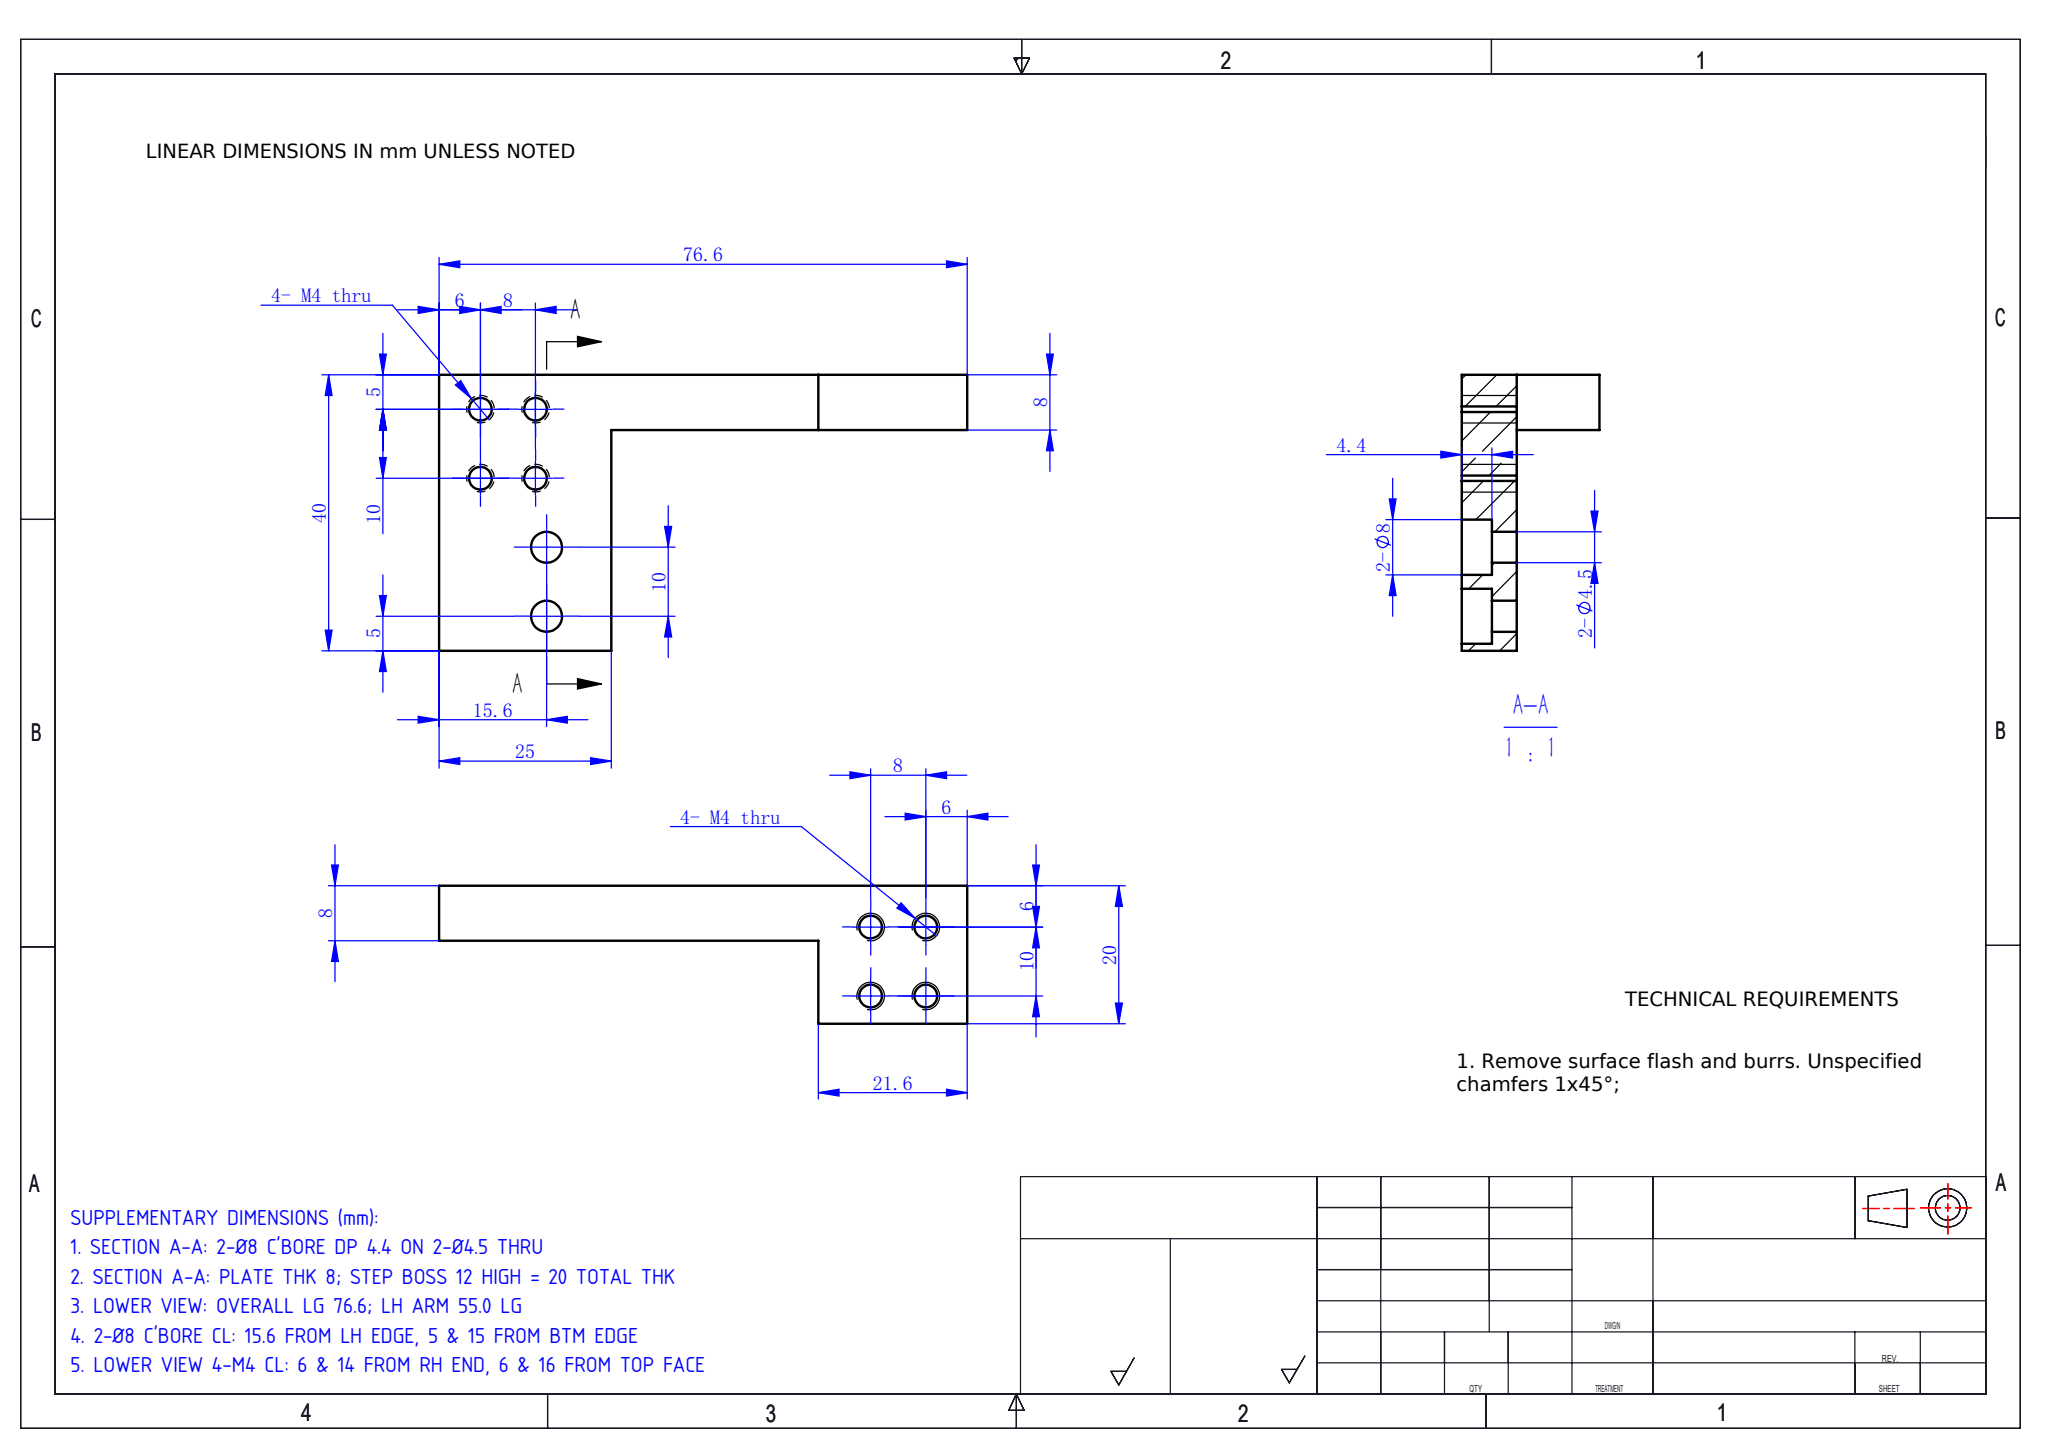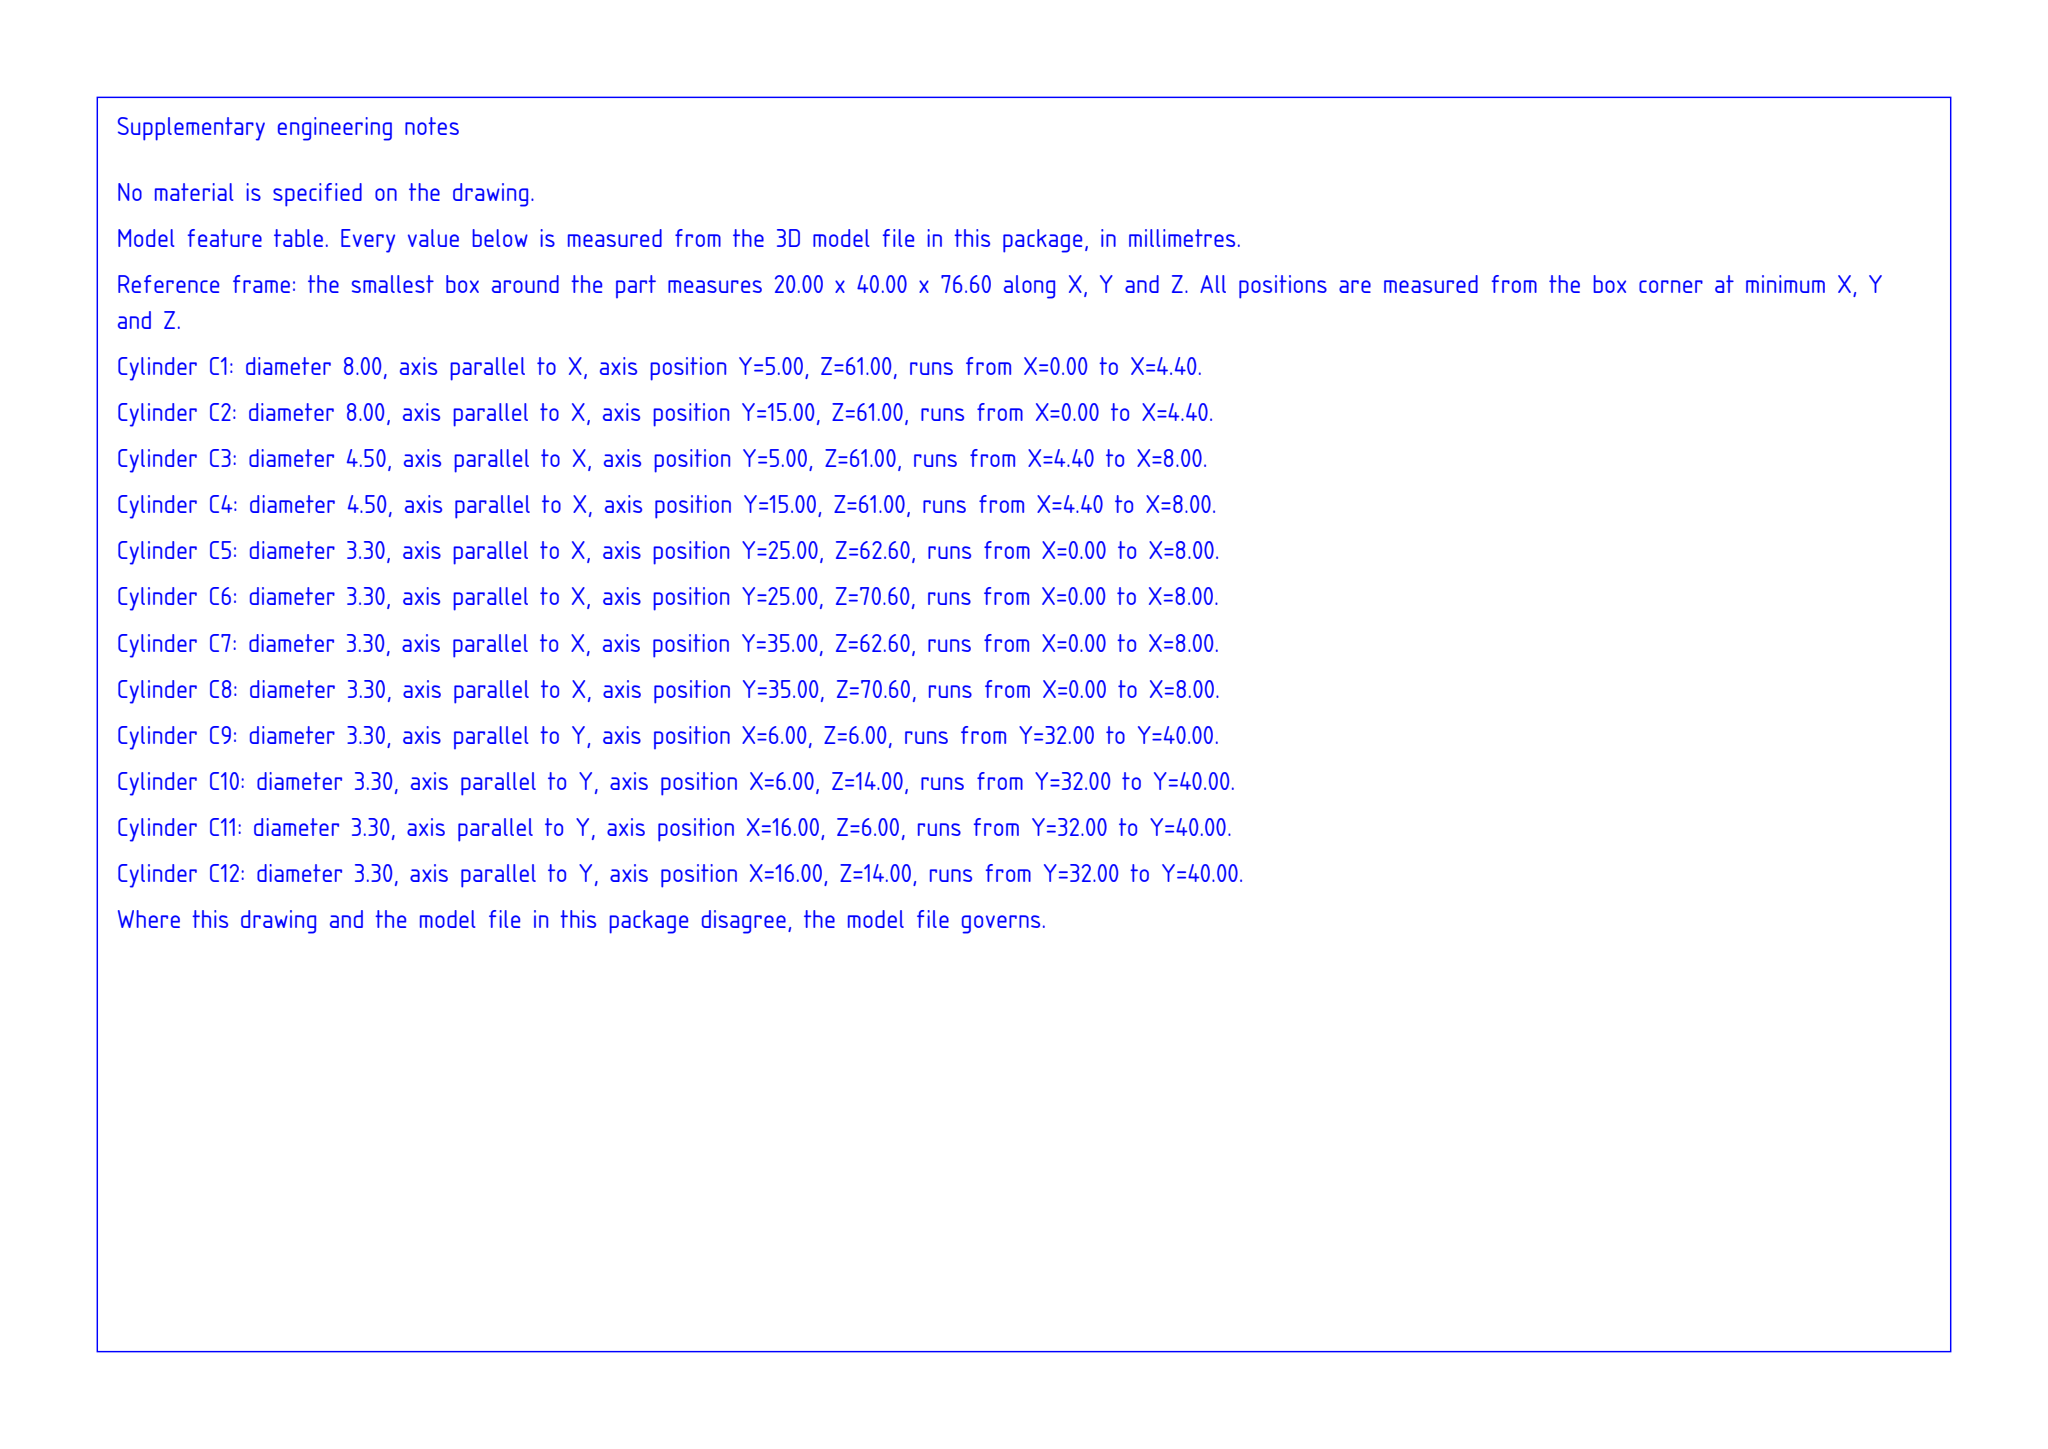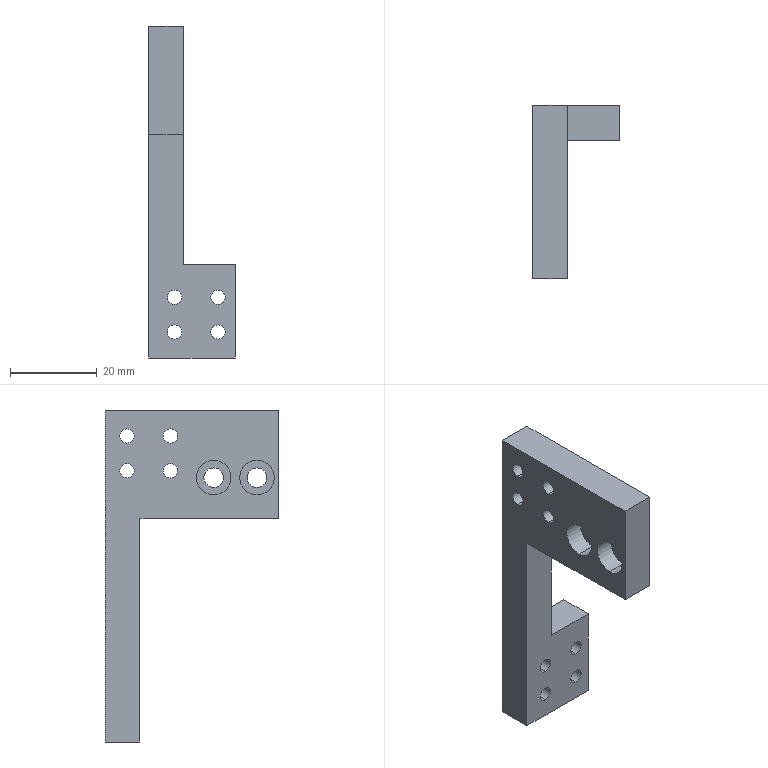Part | SolidWorks | mm | 1 solid | 36 faces | box 20 x 40 x 76.6 mm | volume 12272 mm3 | cylinder 24 | plane 12 | commonest cylinder face diameters 3.3 x16 8 x4 4.5 x4
build123d program:
from build123d import *

# Parameters (mm, degrees)
SKETCH1_W                                       = 20
SKETCH1_H                                       = 76.6
BOSS_EXTRUDE1_DEPTH                             = 40
SKETCH2_W                                       = 12
SKETCH2_H                                       = 32
CUT_EXTRUDE1_DEPTH                              = 87.992
SKETCH3_W                                       = 12
SKETCH3_H                                       = 55
CUT_EXTRUDE2_DEPTH                              = 57.275
M4_TAPPED_HOLE1_D                               = 3.3
M4_TAPPED_HOLE1_DEPTH                           = 11.5
M4_TAPPED_HOLE1_TIP                             = 0.9914
M4_TAPPED_HOLE2_D                               = 3.3
M4_TAPPED_HOLE2_DEPTH                           = 11.5
M4_TAPPED_HOLE2_TIP                             = 0.9914
M4_HEX_SOCKET_HEAD_CAP_SCREW_CBORE1_D           = 4.5
M4_HEX_SOCKET_HEAD_CAP_SCREW_CBORE1_CBORE_D     = 8
M4_HEX_SOCKET_HEAD_CAP_SCREW_CBORE1_CBORE_DEPTH = 4.4
SKETCH10_W                                      = 51.6
SKETCH10_H                                      = 32
CUT_EXTRUDE3_DEPTH                              = 57.665


with BuildPart() as part:
    # Sketch1 → Boss-Extrude1 (new body)
    with BuildSketch(Plane(origin=(0, 0, 0), x_dir=(1, 0, 0), z_dir=(0, 1, 0))):
        Rectangle(SKETCH1_W, SKETCH1_H)
    extrude(amount=BOSS_EXTRUDE1_DEPTH)

    # Sketch2 → Cut-Extrude1 (cut, through all)
    with BuildSketch(Plane.XY.offset(38.3)):
        with Locations((4, 16)):
            Rectangle(SKETCH2_W, SKETCH2_H)
    extrude(amount=-CUT_EXTRUDE1_DEPTH, mode=Mode.SUBTRACT)

    # Sketch3 → Cut-Extrude2 (cut, through all)
    with BuildSketch(Plane(origin=(0, 40, 0), x_dir=(1, 0, 0), z_dir=(0, 1, 0))):
        with Locations((4, -10.8)):
            Rectangle(SKETCH3_W, SKETCH3_H)
    extrude(amount=-CUT_EXTRUDE2_DEPTH, mode=Mode.SUBTRACT)

    # M4 Tapped Hole1
    with Locations(Plane(origin=(0, 40, 0), x_dir=(1, 0, 0), z_dir=(0, 1, 0))):
        with Locations((6, 32.3), (-4, 32.3), (-4, 24.3), (6, 24.3)):
            Hole(M4_TAPPED_HOLE1_D / 2, depth=M4_TAPPED_HOLE1_DEPTH)
            with Locations((0, 0, -(M4_TAPPED_HOLE1_DEPTH + M4_TAPPED_HOLE1_TIP / 2))):  # 118° drill point
                Cone(0, M4_TAPPED_HOLE1_D / 2, M4_TAPPED_HOLE1_TIP, mode=Mode.SUBTRACT)

    # M4 Tapped Hole2
    with Locations(Plane.ZY.offset(10)):
        with Locations((24.3, 35), (24.3, 25), (32.3, 25), (32.3, 35)):
            Hole(M4_TAPPED_HOLE2_D / 2, depth=M4_TAPPED_HOLE2_DEPTH)
            with Locations((0, 0, -(M4_TAPPED_HOLE2_DEPTH + M4_TAPPED_HOLE2_TIP / 2))):  # 118° drill point
                Cone(0, M4_TAPPED_HOLE2_D / 2, M4_TAPPED_HOLE2_TIP, mode=Mode.SUBTRACT)

    # M4 Hex Socket Head Cap Screw CBORE1 (through all)
    with Locations(Plane.ZY.offset(10)):
        with Locations((22.7, 15), (22.7, 5)):
            CounterBoreHole(M4_HEX_SOCKET_HEAD_CAP_SCREW_CBORE1_D / 2, M4_HEX_SOCKET_HEAD_CAP_SCREW_CBORE1_CBORE_D / 2, M4_HEX_SOCKET_HEAD_CAP_SCREW_CBORE1_CBORE_DEPTH)

    # Sketch10 → Cut-Extrude3 (cut, through all)
    with BuildSketch(Plane(origin=(-2, 0, 0), x_dir=(0, 0, -1), z_dir=(1, 0, 0))):
        with Locations((12.5, 16)):
            Rectangle(SKETCH10_W, SKETCH10_H)
    extrude(amount=-CUT_EXTRUDE3_DEPTH, mode=Mode.SUBTRACT)


solid = part.part